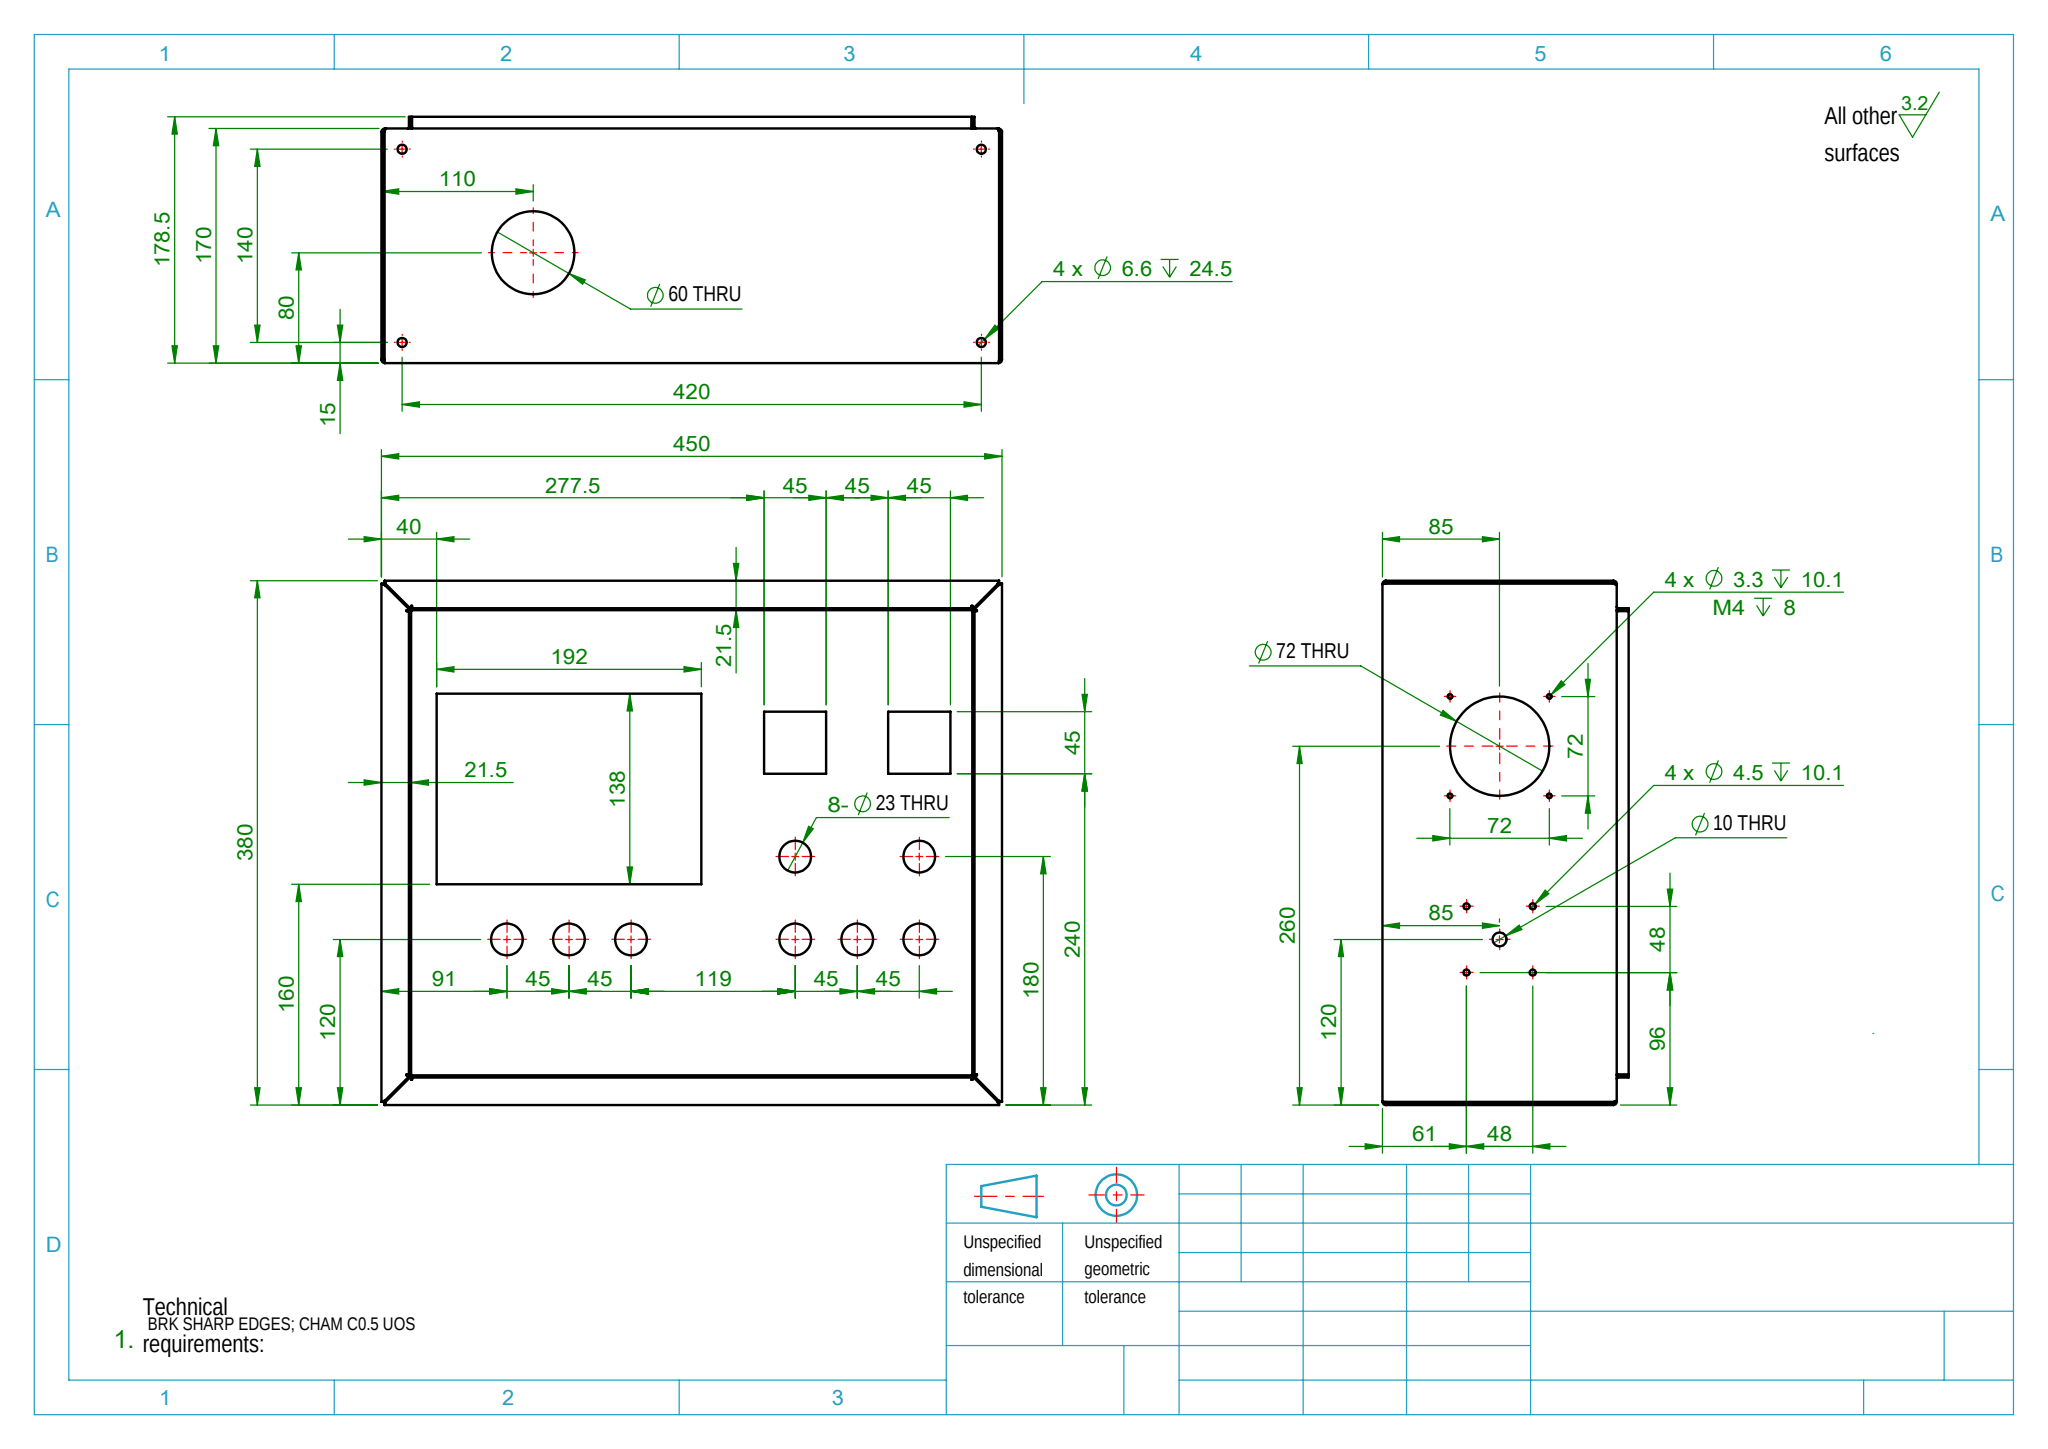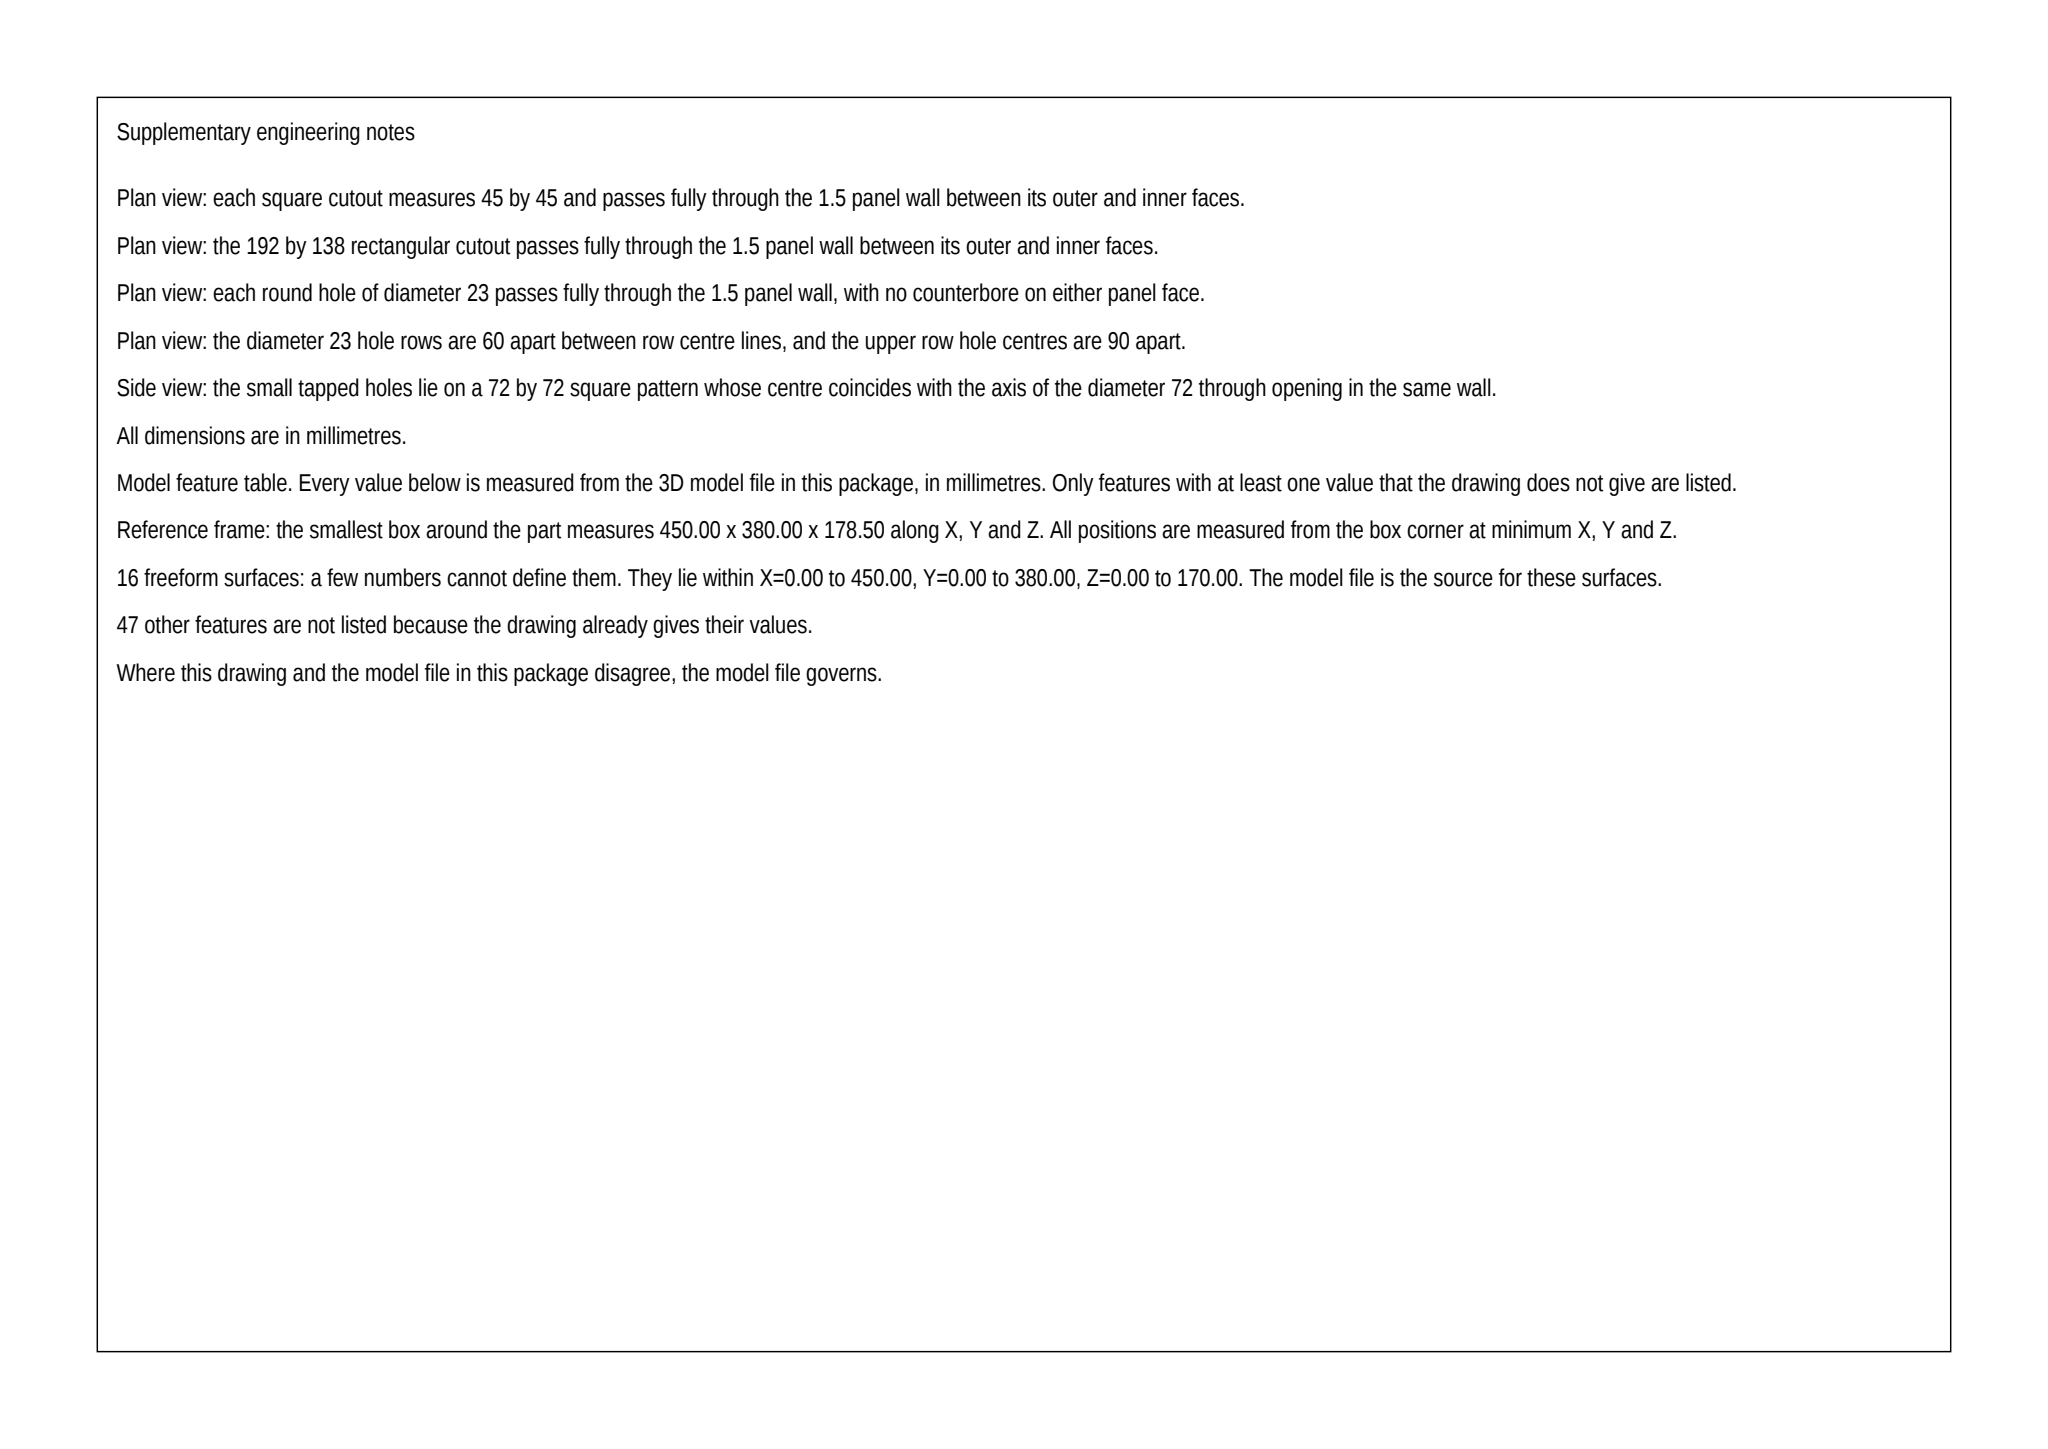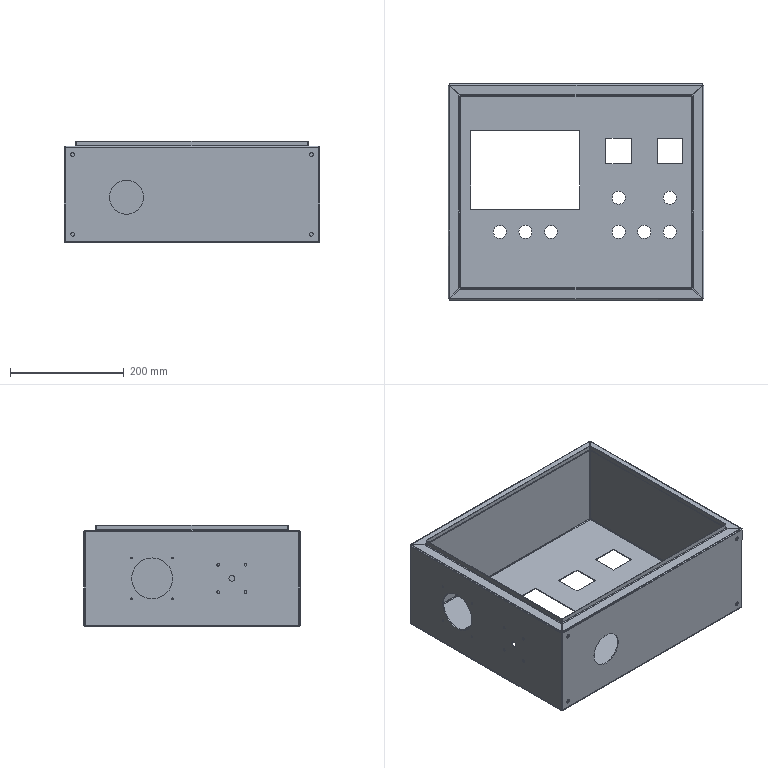Part | SolidWorks | mm | 1 solid | 184 faces | box 450 x 380 x 178.5 mm | volume 670309 mm3 | plane 98 | cylinder 70 | spline 16 | commonest cylinder face diameters 23 x16 5 x12 2 x12 6.6 x8 4.5 x8 3.3 x8 60 x2 10 x2
Drawing notes:
ALL BENDS: INNER R1, OUTER R2.5 (t=1.5) | from the solid: Ø2.0 cyls (R1 inner) and Ø5.0 cyls (R2.5 outer) coaxial at every formed edge, e.g. [2.0,'x',[null,2.52,2.52],445.59] with [5.0,'x',[null,2.52,2.52],445.59]